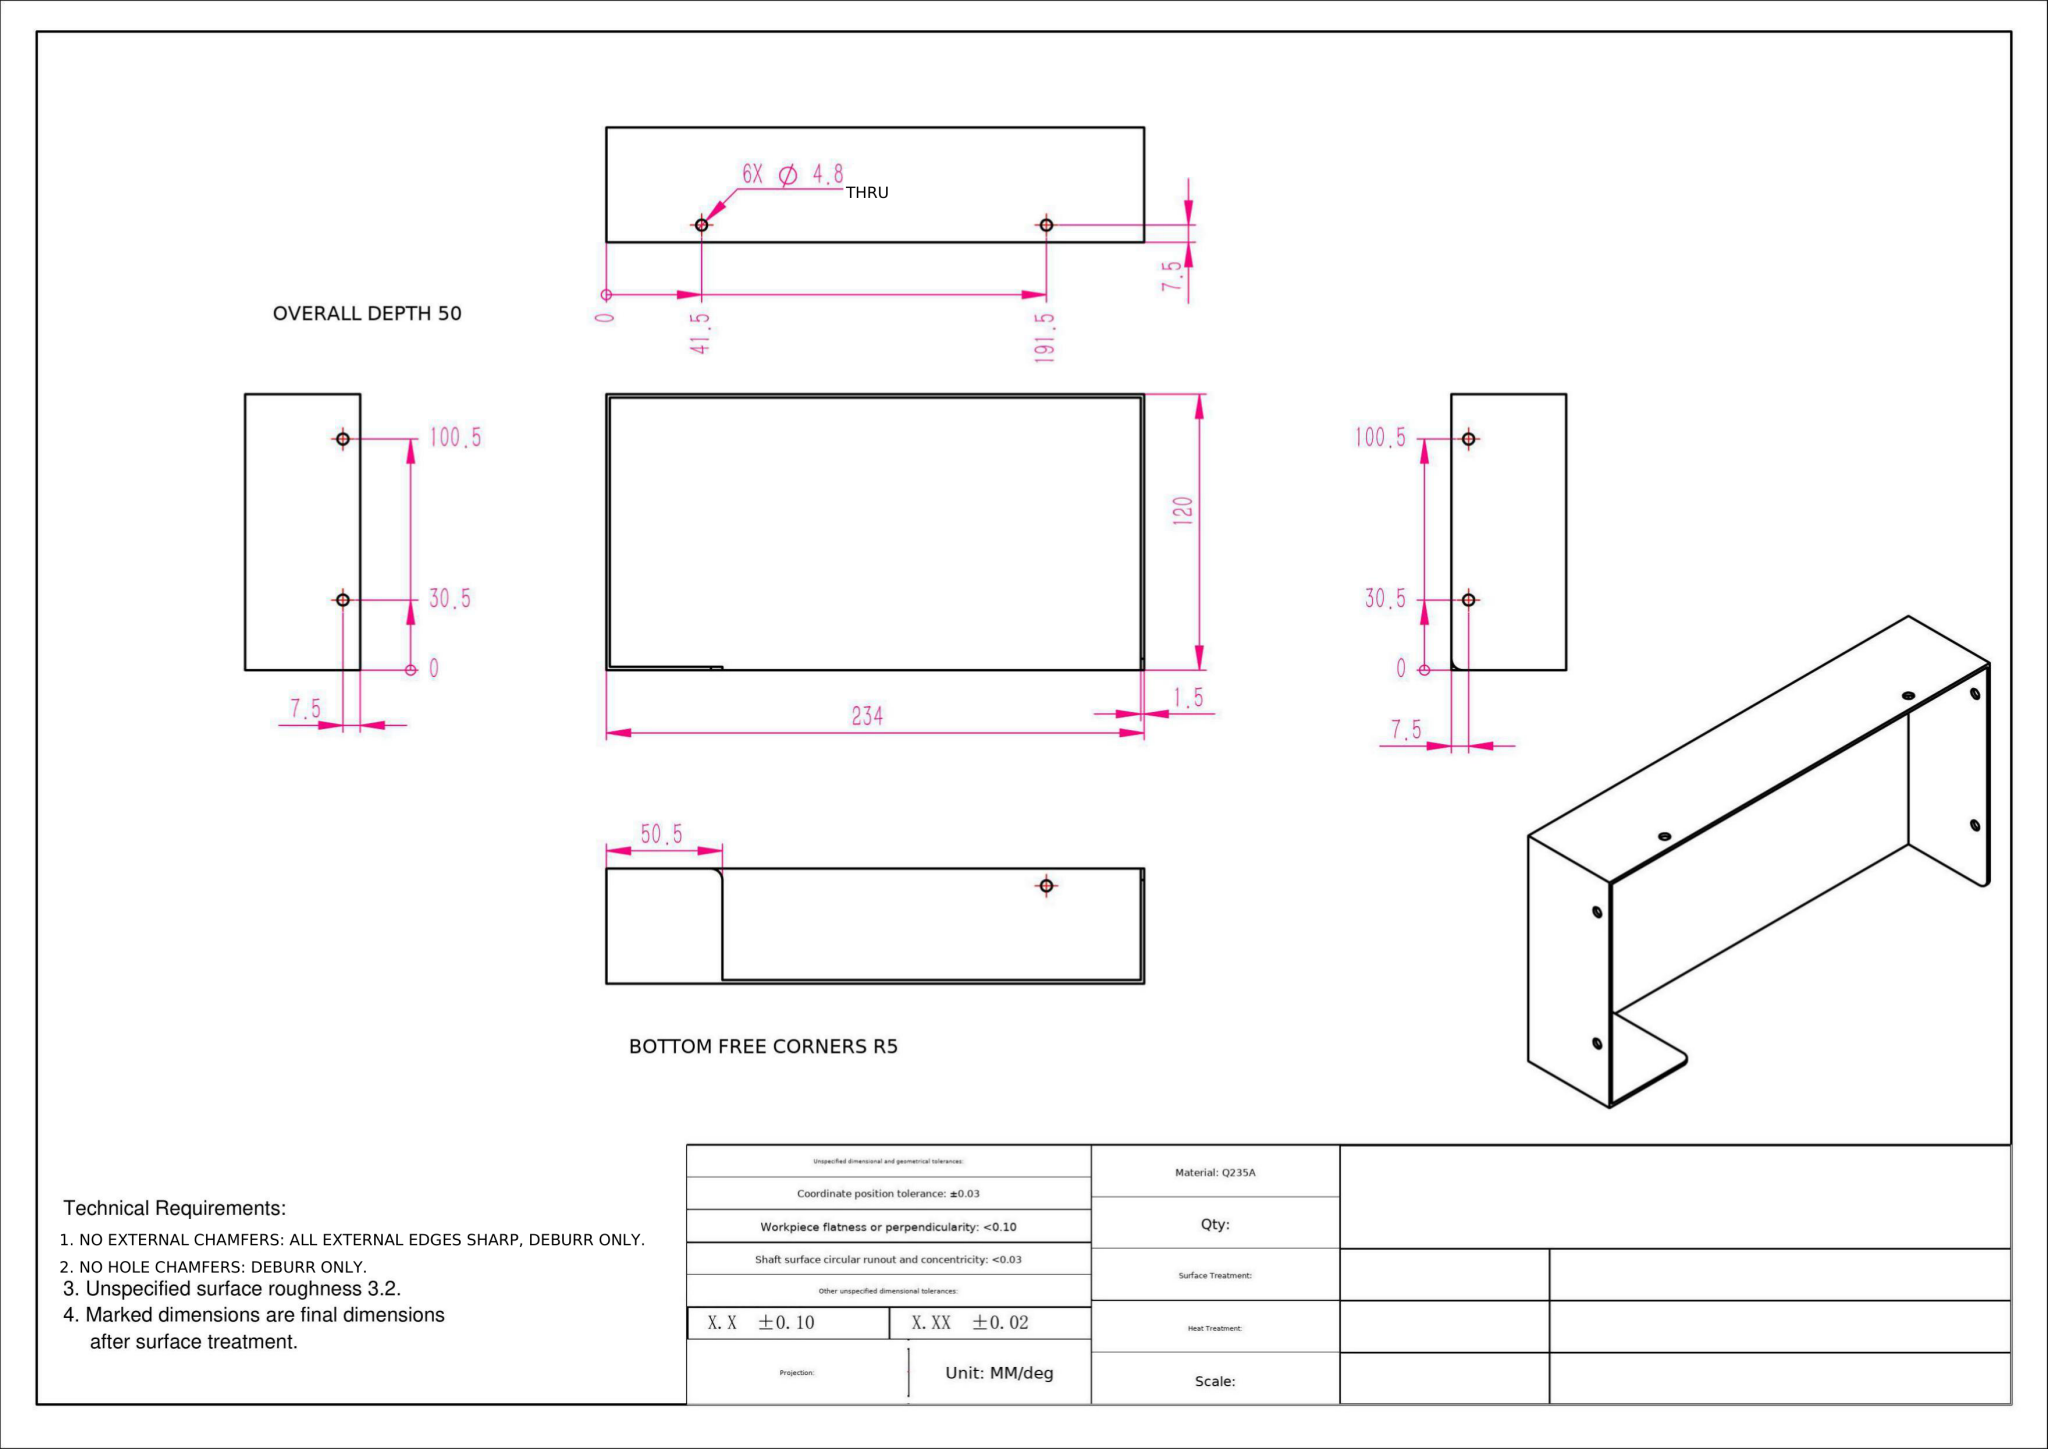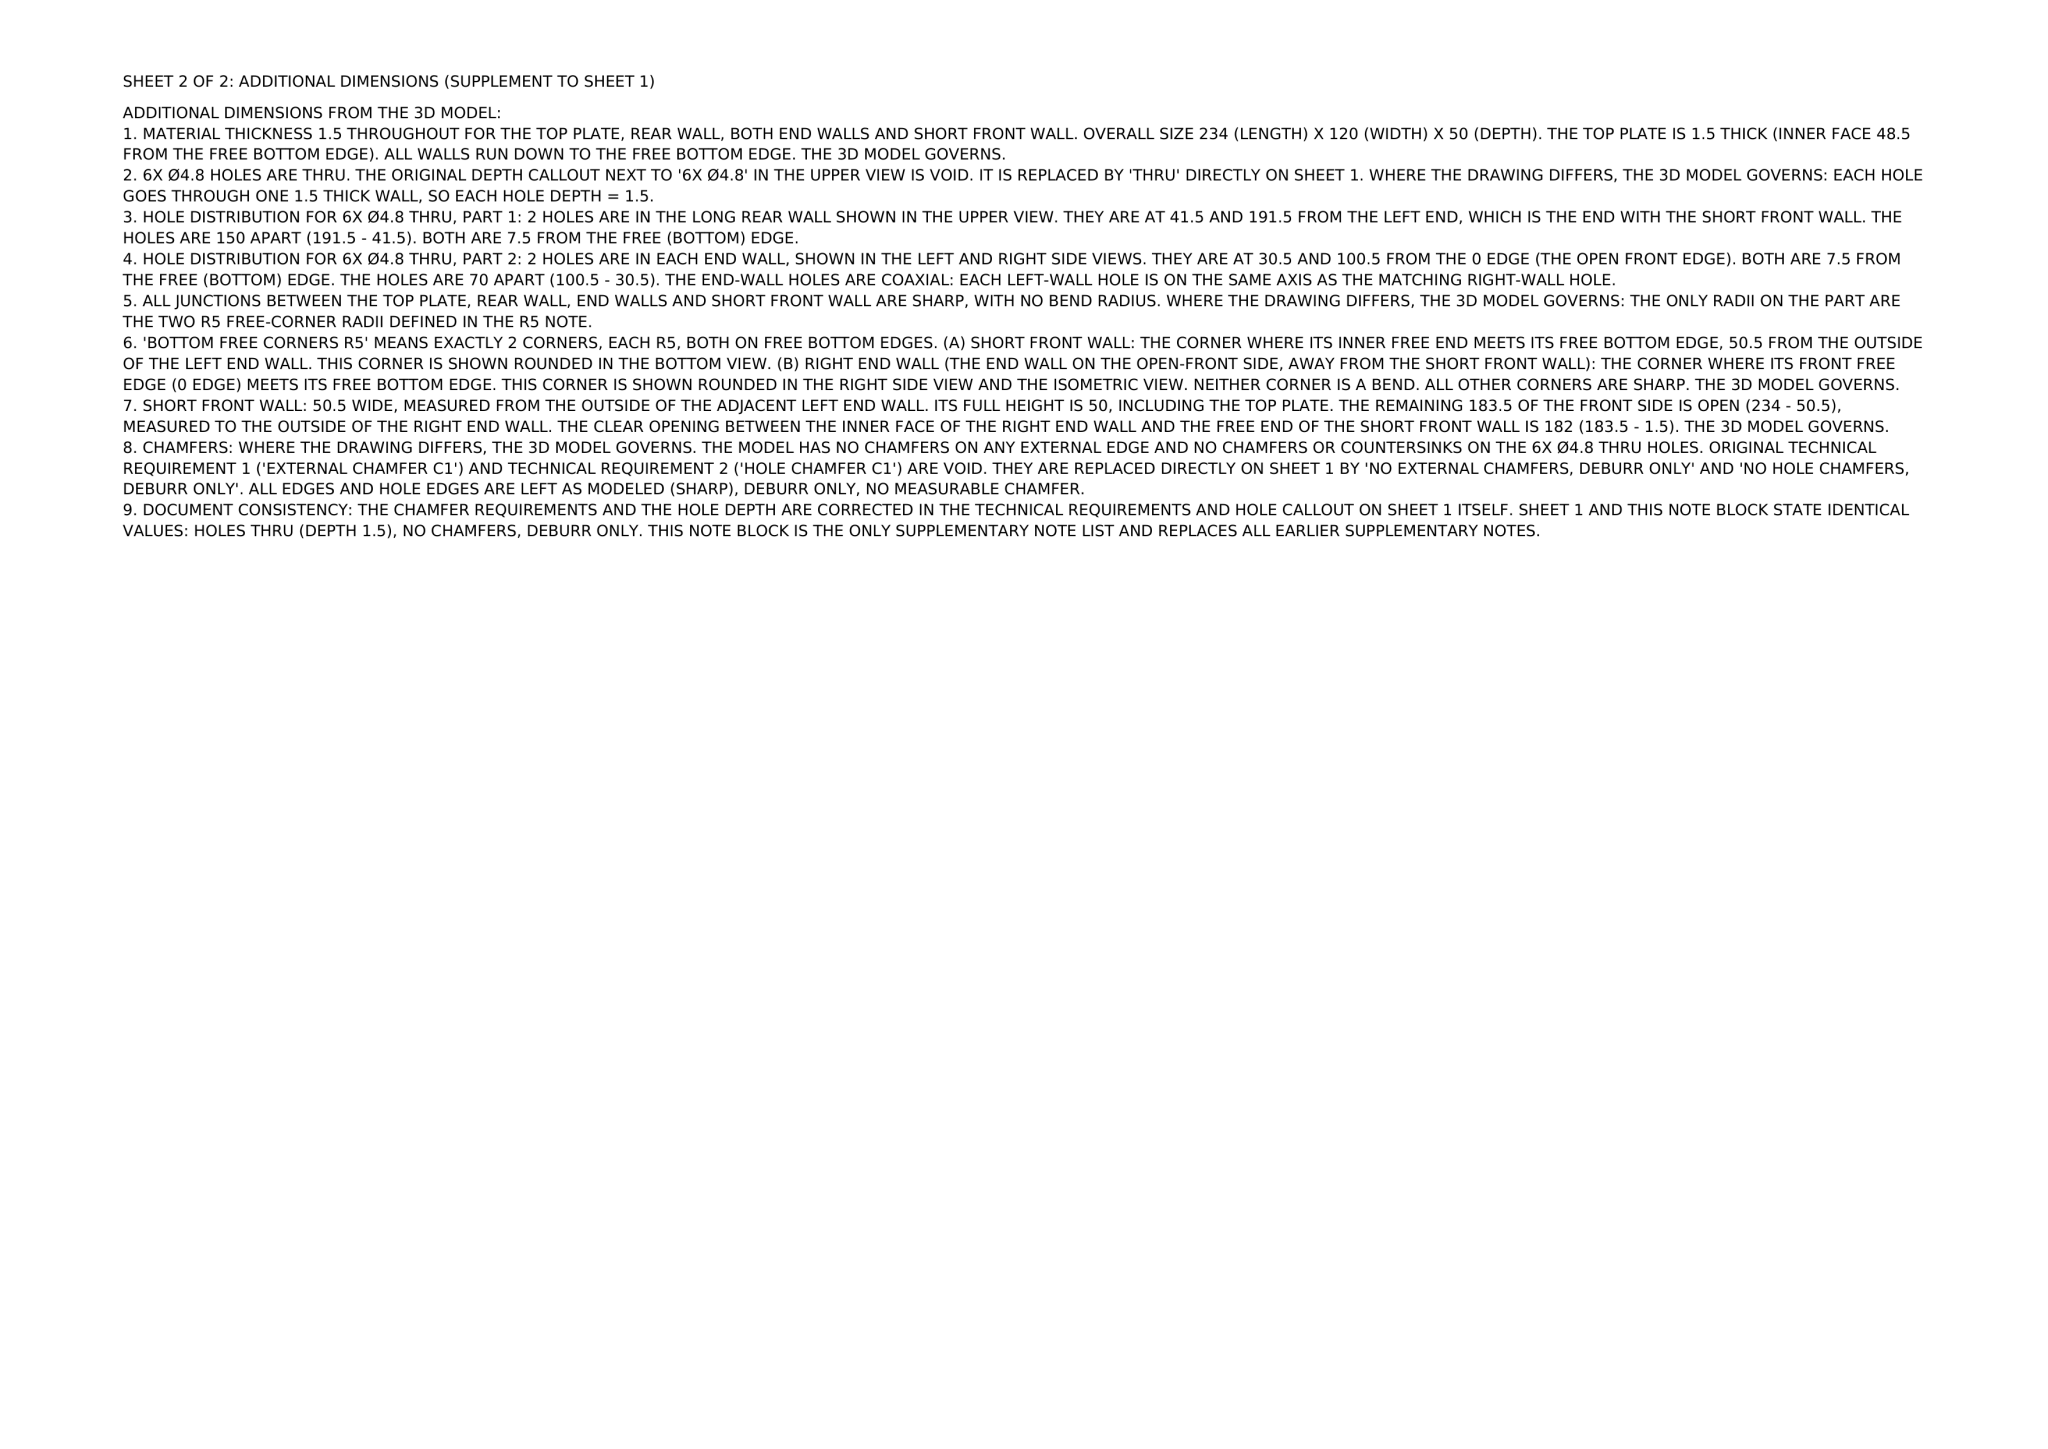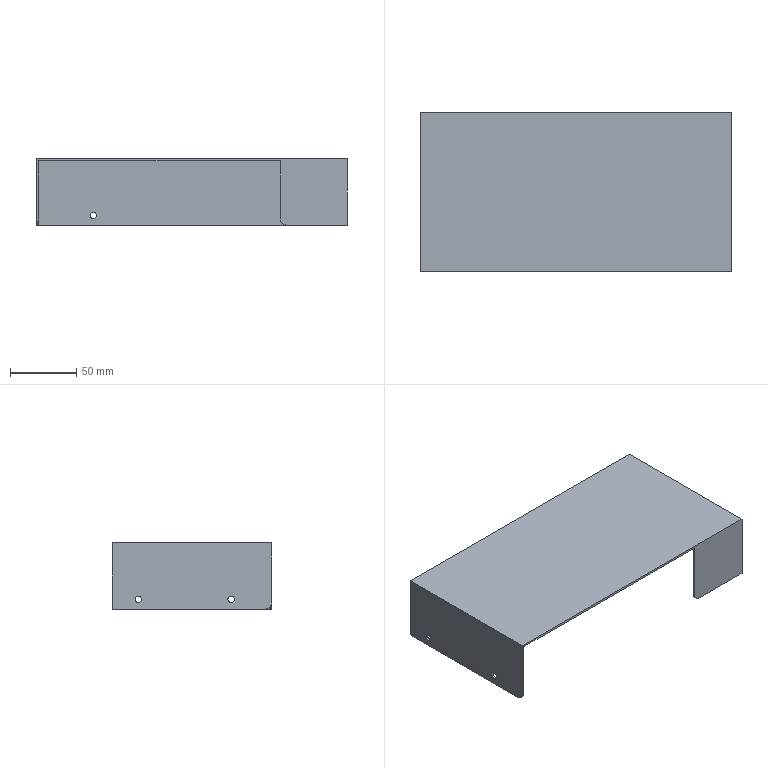Part | NX | mm | Rectangular U-Channel Frame Panel 120mm | 1 solid | 26 faces | box 234 x 120 x 50 mm | volume 79771 mm3 | cylinder 14 | plane 12 | commonest cylinder face diameters 4.8 x12 10 x2
STEP:
#1=COLOUR_RGB('',1.,1.,0.502);
#2=FILL_AREA_STYLE_COLOUR('',#1);
#3=FILL_AREA_STYLE('',(#2));
#4=SURFACE_STYLE_FILL_AREA(#3);
#5=SURFACE_SIDE_STYLE('',(#4));
#6=SURFACE_STYLE_USAGE(.BOTH.,#5);
#7=PRESENTATION_STYLE_ASSIGNMENT((#6));
#8=CARTESIAN_POINT('',(115.5,-29.5,5.1));
#9=VERTEX_POINT('',#8);
#10=CARTESIAN_POINT('',(115.5,-29.5,9.9));
#11=VERTEX_POINT('',#10);
#12=CARTESIAN_POINT('',(115.5,-29.5,7.5));
#13=DIRECTION('',(-1.,0.,0.));
#14=DIRECTION('',(0.,0.,1.));
#15=AXIS2_PLACEMENT_3D('',#12,#13,#14);
#16=CIRCLE('',#15,2.4);
#17=EDGE_CURVE('',#9,#11,#16,.T.);
#18=ORIENTED_EDGE('',*,*,#17,.T.);
#19=CARTESIAN_POINT('',(117.,-29.5,9.9));
#20=VERTEX_POINT('',#19);
#21=CARTESIAN_POINT('',(117.,-29.5,9.9));
#22=DIRECTION('',(1.,0.,0.));
#23=VECTOR('',#22,1000.);
#24=LINE('',#21,#23);
#25=EDGE_CURVE('',#11,#20,#24,.T.);
#26=ORIENTED_EDGE('',*,*,#25,.T.);
#27=CARTESIAN_POINT('',(117.,-29.5,5.1));
#28=VERTEX_POINT('',#27);
#29=CARTESIAN_POINT('',(117.,-29.5,7.5));
#30=DIRECTION('',(1.,0.,0.));
#31=DIRECTION('',(0.,0.,-1.));
#32=AXIS2_PLACEMENT_3D('',#29,#30,#31);
#33=CIRCLE('',#32,2.4);
#34=EDGE_CURVE('',#20,#28,#33,.T.);
#35=ORIENTED_EDGE('',*,*,#34,.T.);
#36=CARTESIAN_POINT('',(117.,-29.5,5.1));
#37=DIRECTION('',(1.,0.,0.));
#38=VECTOR('',#37,1000.);
#39=LINE('',#36,#38);
#40=EDGE_CURVE('',#9,#28,#39,.T.);
#41=ORIENTED_EDGE('',*,*,#40,.F.);
#42=EDGE_LOOP('',(#18,#26,#35,#41));
#43=FACE_OUTER_BOUND('',#42,.T.);
#44=CARTESIAN_POINT('',(117.,-29.5,7.5));
#45=DIRECTION('',(1.,0.,0.));
#46=DIRECTION('',(0.,0.,-1.));
#47=AXIS2_PLACEMENT_3D('',#44,#45,#46);
#48=CYLINDRICAL_SURFACE('',#47,2.4);
#49=ADVANCED_FACE('',(#43),#48,.F.);
#50=CARTESIAN_POINT('',(115.5,40.5,5.1));
#51=VERTEX_POINT('',#50);
#52=CARTESIAN_POINT('',(115.5,40.5,9.9));
#53=VERTEX_POINT('',#52);
#54=CARTESIAN_POINT('',(115.5,40.5,7.5));
#55=DIRECTION('',(-1.,0.,0.));
#56=DIRECTION('',(0.,0.,1.));
#57=AXIS2_PLACEMENT_3D('',#54,#55,#56);
#58=CIRCLE('',#57,2.4);
#59=EDGE_CURVE('',#51,#53,#58,.T.);
#60=ORIENTED_EDGE('',*,*,#59,.T.);
#61=CARTESIAN_POINT('',(117.,40.5,9.9));
#62=VERTEX_POINT('',#61);
#63=CARTESIAN_POINT('',(117.,40.5,9.9));
#64=DIRECTION('',(1.,0.,0.));
#65=VECTOR('',#64,1000.);
#66=LINE('',#63,#65);
#67=EDGE_CURVE('',#53,#62,#66,.T.);
#68=ORIENTED_EDGE('',*,*,#67,.T.);
#69=CARTESIAN_POINT('',(117.,40.5,5.1));
#70=VERTEX_POINT('',#69);
#71=CARTESIAN_POINT('',(117.,40.5,7.5));
#72=DIRECTION('',(1.,0.,0.));
#73=DIRECTION('',(0.,0.,-1.));
#74=AXIS2_PLACEMENT_3D('',#71,#72,#73);
#75=CIRCLE('',#74,2.4);
#76=EDGE_CURVE('',#62,#70,#75,.T.);
#77=ORIENTED_EDGE('',*,*,#76,.T.);
#78=CARTESIAN_POINT('',(117.,40.5,5.1));
#79=DIRECTION('',(1.,0.,0.));
#80=VECTOR('',#79,1000.);
#81=LINE('',#78,#80);
#82=EDGE_CURVE('',#51,#70,#81,.T.);
#83=ORIENTED_EDGE('',*,*,#82,.F.);
#84=EDGE_LOOP('',(#60,#68,#77,#83));
#85=FACE_OUTER_BOUND('',#84,.T.);
#86=CARTESIAN_POINT('',(117.,40.5,7.5));
#87=DIRECTION('',(1.,0.,0.));
#88=DIRECTION('',(0.,0.,-1.));
#89=AXIS2_PLACEMENT_3D('',#86,#87,#88);
#90=CYLINDRICAL_SURFACE('',#89,2.4);
#91=ADVANCED_FACE('',(#85),#90,.F.);
#92=CARTESIAN_POINT('',(75.5,58.5,9.9));
#93=VERTEX_POINT('',#92);
#94=CARTESIAN_POINT('',(75.5,58.5,5.1));
#95=VERTEX_POINT('',#94);
#96=CARTESIAN_POINT('',(75.5,58.5,7.5));
#97=DIRECTION('',(0.,-1.,0.));
#98=DIRECTION('',(0.,0.,-1.));
#99=AXIS2_PLACEMENT_3D('',#96,#97,#98);
#100=CIRCLE('',#99,2.4);
#101=EDGE_CURVE('',#93,#95,#100,.T.);
#102=ORIENTED_EDGE('',*,*,#101,.T.);
#103=CARTESIAN_POINT('',(75.5,60.,5.1));
#104=VERTEX_POINT('',#103);
#105=CARTESIAN_POINT('',(75.5,60.,5.1));
#106=DIRECTION('',(0.,1.,0.));
#107=VECTOR('',#106,1000.);
#108=LINE('',#105,#107);
#109=EDGE_CURVE('',#95,#104,#108,.T.);
#110=ORIENTED_EDGE('',*,*,#109,.T.);
#111=CARTESIAN_POINT('',(75.5,60.,9.9));
#112=VERTEX_POINT('',#111);
#113=CARTESIAN_POINT('',(75.5,60.,7.5));
#114=DIRECTION('',(0.,1.,0.));
#115=DIRECTION('',(0.,0.,1.));
#116=AXIS2_PLACEMENT_3D('',#113,#114,#115);
#117=CIRCLE('',#116,2.4);
#118=EDGE_CURVE('',#104,#112,#117,.T.);
#119=ORIENTED_EDGE('',*,*,#118,.T.);
#120=CARTESIAN_POINT('',(75.5,60.,9.9));
#121=DIRECTION('',(0.,1.,0.));
#122=VECTOR('',#121,1000.);
#123=LINE('',#120,#122);
#124=EDGE_CURVE('',#93,#112,#123,.T.);
#125=ORIENTED_EDGE('',*,*,#124,.F.);
#126=EDGE_LOOP('',(#102,#110,#119,#125));
#127=FACE_OUTER_BOUND('',#126,.T.);
#128=CARTESIAN_POINT('',(75.5,60.,7.5));
#129=DIRECTION('',(0.,1.,0.));
#130=DIRECTION('',(0.,0.,1.));
#131=AXIS2_PLACEMENT_3D('',#128,#129,#130);
#132=CYLINDRICAL_SURFACE('',#131,2.4);
#133=ADVANCED_FACE('',(#127),#132,.F.);
#134=CARTESIAN_POINT('',(-74.5,58.5,9.9));
#135=VERTEX_POINT('',#134);
#136=CARTESIAN_POINT('',(-74.5,58.5,5.1));
#137=VERTEX_POINT('',#136);
#138=CARTESIAN_POINT('',(-74.5,58.5,7.5));
#139=DIRECTION('',(0.,-1.,0.));
#140=DIRECTION('',(0.,0.,-1.));
#141=AXIS2_PLACEMENT_3D('',#138,#139,#140);
#142=CIRCLE('',#141,2.4);
#143=EDGE_CURVE('',#135,#137,#142,.T.);
#144=ORIENTED_EDGE('',*,*,#143,.T.);
#145=CARTESIAN_POINT('',(-74.5,60.,5.1));
#146=VERTEX_POINT('',#145);
#147=CARTESIAN_POINT('',(-74.5,60.,5.1));
#148=DIRECTION('',(0.,1.,0.));
#149=VECTOR('',#148,1000.);
#150=LINE('',#147,#149);
#151=EDGE_CURVE('',#137,#146,#150,.T.);
#152=ORIENTED_EDGE('',*,*,#151,.T.);
#153=CARTESIAN_POINT('',(-74.5,60.,9.9));
#154=VERTEX_POINT('',#153);
#155=CARTESIAN_POINT('',(-74.5,60.,7.5));
#156=DIRECTION('',(0.,1.,0.));
#157=DIRECTION('',(0.,0.,1.));
#158=AXIS2_PLACEMENT_3D('',#155,#156,#157);
#159=CIRCLE('',#158,2.4);
#160=EDGE_CURVE('',#146,#154,#159,.T.);
#161=ORIENTED_EDGE('',*,*,#160,.T.);
#162=CARTESIAN_POINT('',(-74.5,60.,9.9));
#163=DIRECTION('',(0.,1.,0.));
#164=VECTOR('',#163,1000.);
#165=LINE('',#162,#164);
#166=EDGE_CURVE('',#135,#154,#165,.T.);
#167=ORIENTED_EDGE('',*,*,#166,.F.);
#168=EDGE_LOOP('',(#144,#152,#161,#167));
#169=FACE_OUTER_BOUND('',#168,.T.);
#170=CARTESIAN_POINT('',(-74.5,60.,7.5));
#171=DIRECTION('',(0.,1.,0.));
#172=DIRECTION('',(0.,0.,1.));
#173=AXIS2_PLACEMENT_3D('',#170,#171,#172);
#174=CYLINDRICAL_SURFACE('',#173,2.4);
#175=ADVANCED_FACE('',(#169),#174,.F.);
#176=CARTESIAN_POINT('',(-115.5,40.5,9.9));
#177=VERTEX_POINT('',#176);
#178=CARTESIAN_POINT('',(-115.5,40.5,5.1));
#179=VERTEX_POINT('',#178);
#180=CARTESIAN_POINT('',(-115.5,40.5,7.5));
#181=DIRECTION('',(1.,0.,0.));
#182=DIRECTION('',(0.,0.,-1.));
#183=AXIS2_PLACEMENT_3D('',#180,#181,#182);
#184=CIRCLE('',#183,2.4);
#185=EDGE_CURVE('',#177,#179,#184,.T.);
#186=ORIENTED_EDGE('',*,*,#185,.T.);
#187=CARTESIAN_POINT('',(-117.,40.5,5.1));
#188=VERTEX_POINT('',#187);
#189=CARTESIAN_POINT('',(-117.,40.5,5.1));
#190=DIRECTION('',(-1.,0.,0.));
#191=VECTOR('',#190,1000.);
#192=LINE('',#189,#191);
#193=EDGE_CURVE('',#179,#188,#192,.T.);
#194=ORIENTED_EDGE('',*,*,#193,.T.);
#195=CARTESIAN_POINT('',(-117.,40.5,9.9));
#196=VERTEX_POINT('',#195);
#197=CARTESIAN_POINT('',(-117.,40.5,7.5));
#198=DIRECTION('',(-1.,0.,0.));
#199=DIRECTION('',(0.,0.,1.));
#200=AXIS2_PLACEMENT_3D('',#197,#198,#199);
#201=CIRCLE('',#200,2.4);
#202=EDGE_CURVE('',#188,#196,#201,.T.);
#203=ORIENTED_EDGE('',*,*,#202,.T.);
#204=CARTESIAN_POINT('',(-117.,40.5,9.9));
#205=DIRECTION('',(-1.,0.,0.));
#206=VECTOR('',#205,1000.);
#207=LINE('',#204,#206);
#208=EDGE_CURVE('',#177,#196,#207,.T.);
#209=ORIENTED_EDGE('',*,*,#208,.F.);
#210=EDGE_LOOP('',(#186,#194,#203,#209));
#211=FACE_OUTER_BOUND('',#210,.T.);
#212=CARTESIAN_POINT('',(-117.,40.5,7.5));
#213=DIRECTION('',(-1.,0.,0.));
#214=DIRECTION('',(0.,0.,1.));
#215=AXIS2_PLACEMENT_3D('',#212,#213,#214);
#216=CYLINDRICAL_SURFACE('',#215,2.4);
#217=ADVANCED_FACE('',(#211),#216,.F.);
#218=CARTESIAN_POINT('',(-115.5,-29.5,9.9));
#219=VERTEX_POINT('',#218);
#220=CARTESIAN_POINT('',(-115.5,-29.5,5.1));
#221=VERTEX_POINT('',#220);
#222=CARTESIAN_POINT('',(-115.5,-29.5,7.5));
#223=DIRECTION('',(1.,0.,0.));
#224=DIRECTION('',(0.,0.,-1.));
#225=AXIS2_PLACEMENT_3D('',#222,#223,#224);
#226=CIRCLE('',#225,2.4);
#227=EDGE_CURVE('',#219,#221,#226,.T.);
#228=ORIENTED_EDGE('',*,*,#227,.T.);
#229=CARTESIAN_POINT('',(-117.,-29.5,5.1));
#230=VERTEX_POINT('',#229);
#231=CARTESIAN_POINT('',(-117.,-29.5,5.1));
#232=DIRECTION('',(-1.,0.,0.));
#233=VECTOR('',#232,1000.);
#234=LINE('',#231,#233);
#235=EDGE_CURVE('',#221,#230,#234,.T.);
#236=ORIENTED_EDGE('',*,*,#235,.T.);
#237=CARTESIAN_POINT('',(-117.,-29.5,9.9));
#238=VERTEX_POINT('',#237);
#239=CARTESIAN_POINT('',(-117.,-29.5,7.5));
#240=DIRECTION('',(-1.,0.,0.));
#241=DIRECTION('',(0.,0.,1.));
#242=AXIS2_PLACEMENT_3D('',#239,#240,#241);
#243=CIRCLE('',#242,2.4);
#244=EDGE_CURVE('',#230,#238,#243,.T.);
#245=ORIENTED_EDGE('',*,*,#244,.T.);
#246=CARTESIAN_POINT('',(-117.,-29.5,9.9));
#247=DIRECTION('',(-1.,0.,0.));
#248=VECTOR('',#247,1000.);
#249=LINE('',#246,#248);
#250=EDGE_CURVE('',#219,#238,#249,.T.);
#251=ORIENTED_EDGE('',*,*,#250,.F.);
#252=EDGE_LOOP('',(#228,#236,#245,#251));
#253=FACE_OUTER_BOUND('',#252,.T.);
#254=CARTESIAN_POINT('',(-117.,-29.5,7.5));
#255=DIRECTION('',(-1.,0.,0.));
#256=DIRECTION('',(0.,0.,1.));
#257=AXIS2_PLACEMENT_3D('',#254,#255,#256);
#258=CYLINDRICAL_SURFACE('',#257,2.4);
#259=ADVANCED_FACE('',(#253),#258,.F.);
#260=CARTESIAN_POINT('',(71.5,-60.,0.));
#261=VERTEX_POINT('',#260);
#262=CARTESIAN_POINT('',(117.,-60.,0.));
#263=VERTEX_POINT('',#262);
#264=CARTESIAN_POINT('',(-117.,-60.,0.));
#265=DIRECTION('',(1.,0.,0.));
#266=VECTOR('',#265,1000.);
#267=LINE('',#264,#266);
#268=EDGE_CURVE('',#261,#263,#267,.T.);
#269=ORIENTED_EDGE('',*,*,#268,.F.);
#270=CARTESIAN_POINT('',(71.5,-58.5,0.));
#271=VERTEX_POINT('',#270);
#272=CARTESIAN_POINT('',(71.5,-58.5,0.));
#273=DIRECTION('',(0.,1.,0.));
#274=VECTOR('',#273,1000.);
#275=LINE('',#272,#274);
#276=EDGE_CURVE('',#261,#271,#275,.T.);
#277=ORIENTED_EDGE('',*,*,#276,.T.);
#278=CARTESIAN_POINT('',(115.5,-58.5,0.));
#279=VERTEX_POINT('',#278);
#280=CARTESIAN_POINT('',(0.,-58.5,0.));
#281=DIRECTION('',(1.,0.,0.));
#282=VECTOR('',#281,1000.);
#283=LINE('',#280,#282);
#284=EDGE_CURVE('',#271,#279,#283,.T.);
#285=ORIENTED_EDGE('',*,*,#284,.T.);
#286=CARTESIAN_POINT('',(115.5,58.5,0.));
#287=VERTEX_POINT('',#286);
#288=CARTESIAN_POINT('',(115.5,0.,0.));
#289=DIRECTION('',(0.,1.,0.));
#290=VECTOR('',#289,1000.);
#291=LINE('',#288,#290);
#292=EDGE_CURVE('',#279,#287,#291,.T.);
#293=ORIENTED_EDGE('',*,*,#292,.T.);
#294=CARTESIAN_POINT('',(-115.5,58.5,0.));
#295=VERTEX_POINT('',#294);
#296=CARTESIAN_POINT('',(0.,58.5,0.));
#297=DIRECTION('',(-1.,0.,0.));
#298=VECTOR('',#297,1000.);
#299=LINE('',#296,#298);
#300=EDGE_CURVE('',#287,#295,#299,.T.);
#301=ORIENTED_EDGE('',*,*,#300,.T.);
#302=CARTESIAN_POINT('',(-115.5,-55.,0.));
#303=VERTEX_POINT('',#302);
#304=CARTESIAN_POINT('',(-115.5,0.,0.));
#305=DIRECTION('',(0.,-1.,0.));
#306=VECTOR('',#305,1000.);
#307=LINE('',#304,#306);
#308=EDGE_CURVE('',#295,#303,#307,.T.);
#309=ORIENTED_EDGE('',*,*,#308,.T.);
#310=CARTESIAN_POINT('',(-117.,-55.,0.));
#311=VERTEX_POINT('',#310);
#312=CARTESIAN_POINT('',(-117.,-55.,0.));
#313=DIRECTION('',(-1.,0.,0.));
#314=VECTOR('',#313,1000.);
#315=LINE('',#312,#314);
#316=EDGE_CURVE('',#303,#311,#315,.T.);
#317=ORIENTED_EDGE('',*,*,#316,.T.);
#318=CARTESIAN_POINT('',(-117.,60.,0.));
#319=VERTEX_POINT('',#318);
#320=CARTESIAN_POINT('',(-117.,-60.,0.));
#321=DIRECTION('',(0.,-1.,0.));
#322=VECTOR('',#321,1000.);
#323=LINE('',#320,#322);
#324=EDGE_CURVE('',#319,#311,#323,.T.);
#325=ORIENTED_EDGE('',*,*,#324,.F.);
#326=CARTESIAN_POINT('',(117.,60.,0.));
#327=VERTEX_POINT('',#326);
#328=CARTESIAN_POINT('',(-117.,60.,0.));
#329=DIRECTION('',(-1.,0.,0.));
#330=VECTOR('',#329,1000.);
#331=LINE('',#328,#330);
#332=EDGE_CURVE('',#327,#319,#331,.T.);
#333=ORIENTED_EDGE('',*,*,#332,.F.);
#334=CARTESIAN_POINT('',(117.,-60.,0.));
#335=DIRECTION('',(0.,1.,0.));
#336=VECTOR('',#335,1000.);
#337=LINE('',#334,#336);
#338=EDGE_CURVE('',#263,#327,#337,.T.);
#339=ORIENTED_EDGE('',*,*,#338,.F.);
#340=EDGE_LOOP('',(#269,#277,#285,#293,#301,#309,#317,#325,#333,#339));
#341=FACE_OUTER_BOUND('',#340,.T.);
#342=CARTESIAN_POINT('',(0.,0.,0.));
#343=DIRECTION('',(0.,0.,-1.));
#344=DIRECTION('',(-1.,0.,0.));
#345=AXIS2_PLACEMENT_3D('',#342,#343,#344);
#346=PLANE('',#345);
#347=ADVANCED_FACE('',(#341),#346,.T.);
#348=CARTESIAN_POINT('',(117.,-29.5,7.5));
#349=DIRECTION('',(1.,0.,0.));
#350=DIRECTION('',(0.,0.,-1.));
#351=AXIS2_PLACEMENT_3D('',#348,#349,#350);
#352=CIRCLE('',#351,2.4);
#353=EDGE_CURVE('',#28,#20,#352,.T.);
#354=ORIENTED_EDGE('',*,*,#353,.F.);
#355=ORIENTED_EDGE('',*,*,#34,.F.);
#356=EDGE_LOOP('',(#354,#355));
#357=FACE_BOUND('',#356,.T.);
#358=CARTESIAN_POINT('',(117.,40.5,7.5));
#359=DIRECTION('',(1.,0.,0.));
#360=DIRECTION('',(0.,0.,-1.));
#361=AXIS2_PLACEMENT_3D('',#358,#359,#360);
#362=CIRCLE('',#361,2.4);
#363=EDGE_CURVE('',#70,#62,#362,.T.);
#364=ORIENTED_EDGE('',*,*,#363,.F.);
#365=ORIENTED_EDGE('',*,*,#76,.F.);
#366=EDGE_LOOP('',(#364,#365));
#367=FACE_BOUND('',#366,.T.);
#368=ORIENTED_EDGE('',*,*,#338,.T.);
#369=CARTESIAN_POINT('',(117.,60.,50.));
#370=VERTEX_POINT('',#369);
#371=CARTESIAN_POINT('',(117.,60.,50.));
#372=DIRECTION('',(0.,0.,-1.));
#373=VECTOR('',#372,1000.);
#374=LINE('',#371,#373);
#375=EDGE_CURVE('',#370,#327,#374,.T.);
#376=ORIENTED_EDGE('',*,*,#375,.F.);
#377=CARTESIAN_POINT('',(117.,-60.,50.));
#378=VERTEX_POINT('',#377);
#379=CARTESIAN_POINT('',(117.,-60.,50.));
#380=DIRECTION('',(0.,1.,0.));
#381=VECTOR('',#380,1000.);
#382=LINE('',#379,#381);
#383=EDGE_CURVE('',#378,#370,#382,.T.);
#384=ORIENTED_EDGE('',*,*,#383,.F.);
#385=CARTESIAN_POINT('',(117.,-60.,50.));
#386=DIRECTION('',(0.,0.,-1.));
#387=VECTOR('',#386,1000.);
#388=LINE('',#385,#387);
#389=EDGE_CURVE('',#378,#263,#388,.T.);
#390=ORIENTED_EDGE('',*,*,#389,.T.);
#391=EDGE_LOOP('',(#368,#376,#384,#390));
#392=FACE_OUTER_BOUND('',#391,.T.);
#393=CARTESIAN_POINT('',(117.,-60.,50.));
#394=DIRECTION('',(-1.,0.,0.));
#395=DIRECTION('',(0.,0.,1.));
#396=AXIS2_PLACEMENT_3D('',#393,#394,#395);
#397=PLANE('',#396);
#398=ADVANCED_FACE('',(#357,#367,#392),#397,.F.);
#399=CARTESIAN_POINT('',(75.5,60.,7.5));
#400=DIRECTION('',(0.,1.,0.));
#401=DIRECTION('',(0.,0.,1.));
#402=AXIS2_PLACEMENT_3D('',#399,#400,#401);
#403=CIRCLE('',#402,2.4);
#404=EDGE_CURVE('',#112,#104,#403,.T.);
#405=ORIENTED_EDGE('',*,*,#404,.F.);
#406=ORIENTED_EDGE('',*,*,#118,.F.);
#407=EDGE_LOOP('',(#405,#406));
#408=FACE_BOUND('',#407,.T.);
#409=CARTESIAN_POINT('',(-74.5,60.,7.5));
#410=DIRECTION('',(0.,1.,0.));
#411=DIRECTION('',(0.,0.,1.));
#412=AXIS2_PLACEMENT_3D('',#409,#410,#411);
#413=CIRCLE('',#412,2.4);
#414=EDGE_CURVE('',#154,#146,#413,.T.);
#415=ORIENTED_EDGE('',*,*,#414,.F.);
#416=ORIENTED_EDGE('',*,*,#160,.F.);
#417=EDGE_LOOP('',(#415,#416));
#418=FACE_BOUND('',#417,.T.);
#419=ORIENTED_EDGE('',*,*,#332,.T.);
#420=CARTESIAN_POINT('',(-117.,60.,50.));
#421=VERTEX_POINT('',#420);
#422=CARTESIAN_POINT('',(-117.,60.,50.));
#423=DIRECTION('',(0.,0.,-1.));
#424=VECTOR('',#423,1000.);
#425=LINE('',#422,#424);
#426=EDGE_CURVE('',#421,#319,#425,.T.);
#427=ORIENTED_EDGE('',*,*,#426,.F.);
#428=CARTESIAN_POINT('',(-117.,60.,50.));
#429=DIRECTION('',(-1.,0.,0.));
#430=VECTOR('',#429,1000.);
#431=LINE('',#428,#430);
#432=EDGE_CURVE('',#370,#421,#431,.T.);
#433=ORIENTED_EDGE('',*,*,#432,.F.);
#434=ORIENTED_EDGE('',*,*,#375,.T.);
#435=EDGE_LOOP('',(#419,#427,#433,#434));
#436=FACE_OUTER_BOUND('',#435,.T.);
#437=CARTESIAN_POINT('',(-117.,60.,50.));
#438=DIRECTION('',(0.,-1.,0.));
#439=DIRECTION('',(0.,0.,-1.));
#440=AXIS2_PLACEMENT_3D('',#437,#438,#439);
#441=PLANE('',#440);
#442=ADVANCED_FACE('',(#408,#418,#436),#441,.F.);
#443=CARTESIAN_POINT('',(-117.,40.5,7.5));
#444=DIRECTION('',(-1.,0.,0.));
#445=DIRECTION('',(0.,0.,1.));
#446=AXIS2_PLACEMENT_3D('',#443,#444,#445);
#447=CIRCLE('',#446,2.4);
#448=EDGE_CURVE('',#196,#188,#447,.T.);
#449=ORIENTED_EDGE('',*,*,#448,.F.);
#450=ORIENTED_EDGE('',*,*,#202,.F.);
#451=EDGE_LOOP('',(#449,#450));
#452=FACE_BOUND('',#451,.T.);
#453=CARTESIAN_POINT('',(-117.,-29.5,7.5));
#454=DIRECTION('',(-1.,0.,0.));
#455=DIRECTION('',(0.,0.,1.));
#456=AXIS2_PLACEMENT_3D('',#453,#454,#455);
#457=CIRCLE('',#456,2.4);
#458=EDGE_CURVE('',#238,#230,#457,.T.);
#459=ORIENTED_EDGE('',*,*,#458,.F.);
#460=ORIENTED_EDGE('',*,*,#244,.F.);
#461=EDGE_LOOP('',(#459,#460));
#462=FACE_BOUND('',#461,.T.);
#463=ORIENTED_EDGE('',*,*,#324,.T.);
#464=CARTESIAN_POINT('',(-117.,-60.,5.));
#465=VERTEX_POINT('',#464);
#466=CARTESIAN_POINT('',(-117.,-55.,5.));
#467=DIRECTION('',(-1.,0.,0.));
#468=DIRECTION('',(0.,0.,-1.));
#469=AXIS2_PLACEMENT_3D('',#466,#467,#468);
#470=CIRCLE('',#469,5.);
#471=EDGE_CURVE('',#311,#465,#470,.T.);
#472=ORIENTED_EDGE('',*,*,#471,.T.);
#473=CARTESIAN_POINT('',(-117.,-60.,50.));
#474=VERTEX_POINT('',#473);
#475=CARTESIAN_POINT('',(-117.,-60.,50.));
#476=DIRECTION('',(0.,0.,-1.));
#477=VECTOR('',#476,1000.);
#478=LINE('',#475,#477);
#479=EDGE_CURVE('',#474,#465,#478,.T.);
#480=ORIENTED_EDGE('',*,*,#479,.F.);
#481=CARTESIAN_POINT('',(-117.,-60.,50.));
#482=DIRECTION('',(0.,-1.,0.));
#483=VECTOR('',#482,1000.);
#484=LINE('',#481,#483);
#485=EDGE_CURVE('',#421,#474,#484,.T.);
#486=ORIENTED_EDGE('',*,*,#485,.F.);
#487=ORIENTED_EDGE('',*,*,#426,.T.);
#488=EDGE_LOOP('',(#463,#472,#480,#486,#487));
#489=FACE_OUTER_BOUND('',#488,.T.);
#490=CARTESIAN_POINT('',(-117.,-60.,50.));
#491=DIRECTION('',(1.,0.,0.));
#492=DIRECTION('',(0.,0.,-1.));
#493=AXIS2_PLACEMENT_3D('',#490,#491,#492);
#494=PLANE('',#493);
#495=ADVANCED_FACE('',(#452,#462,#489),#494,.F.);
#496=CARTESIAN_POINT('',(66.5,-60.,5.));
#497=VERTEX_POINT('',#496);
#498=CARTESIAN_POINT('',(66.5,-60.,48.5));
#499=VERTEX_POINT('',#498);
#500=CARTESIAN_POINT('',(66.5,-60.,0.));
#501=DIRECTION('',(0.,0.,1.));
#502=VECTOR('',#501,1000.);
#503=LINE('',#500,#502);
#504=EDGE_CURVE('',#497,#499,#503,.T.);
#505=ORIENTED_EDGE('',*,*,#504,.F.);
#506=CARTESIAN_POINT('',(71.5,-60.,5.));
#507=DIRECTION('',(0.,-1.,0.));
#508=DIRECTION('',(0.,0.,1.));
#509=AXIS2_PLACEMENT_3D('',#506,#507,#508);
#510=CIRCLE('',#509,5.);
#511=EDGE_CURVE('',#497,#261,#510,.T.);
#512=ORIENTED_EDGE('',*,*,#511,.T.);
#513=ORIENTED_EDGE('',*,*,#268,.T.);
#514=ORIENTED_EDGE('',*,*,#389,.F.);
#515=CARTESIAN_POINT('',(-117.,-60.,50.));
#516=DIRECTION('',(1.,0.,0.));
#517=VECTOR('',#516,1000.);
#518=LINE('',#515,#517);
#519=EDGE_CURVE('',#474,#378,#518,.T.);
#520=ORIENTED_EDGE('',*,*,#519,.F.);
#521=ORIENTED_EDGE('',*,*,#479,.T.);
#522=CARTESIAN_POINT('',(-115.5,-60.,5.));
#523=VERTEX_POINT('',#522);
#524=CARTESIAN_POINT('',(-115.5,-60.,5.));
#525=DIRECTION('',(1.,0.,0.));
#526=VECTOR('',#525,1000.);
#527=LINE('',#524,#526);
#528=EDGE_CURVE('',#465,#523,#527,.T.);
#529=ORIENTED_EDGE('',*,*,#528,.T.);
#530=CARTESIAN_POINT('',(-115.5,-60.,48.5));
#531=VERTEX_POINT('',#530);
#532=CARTESIAN_POINT('',(-115.5,-60.,-0.));
#533=DIRECTION('',(0.,0.,-1.));
#534=VECTOR('',#533,1000.);
#535=LINE('',#532,#534);
#536=EDGE_CURVE('',#531,#523,#535,.T.);
#537=ORIENTED_EDGE('',*,*,#536,.F.);
#538=CARTESIAN_POINT('',(66.5,-60.,48.5));
#539=DIRECTION('',(-1.,0.,-0.));
#540=VECTOR('',#539,1000.);
#541=LINE('',#538,#540);
#542=EDGE_CURVE('',#499,#531,#541,.T.);
#543=ORIENTED_EDGE('',*,*,#542,.F.);
#544=EDGE_LOOP('',(#505,#512,#513,#514,#520,#521,#529,#537,#543));
#545=FACE_OUTER_BOUND('',#544,.T.);
#546=CARTESIAN_POINT('',(-117.,-60.,50.));
#547=DIRECTION('',(0.,1.,0.));
#548=DIRECTION('',(0.,0.,1.));
#549=AXIS2_PLACEMENT_3D('',#546,#547,#548);
#550=PLANE('',#549);
#551=ADVANCED_FACE('',(#545),#550,.F.);
#552=ORIENTED_EDGE('',*,*,#383,.T.);
#553=ORIENTED_EDGE('',*,*,#432,.T.);
#554=ORIENTED_EDGE('',*,*,#485,.T.);
#555=ORIENTED_EDGE('',*,*,#519,.T.);
#556=EDGE_LOOP('',(#552,#553,#554,#555));
#557=FACE_OUTER_BOUND('',#556,.T.);
#558=CARTESIAN_POINT('',(0.,0.,50.));
#559=DIRECTION('',(0.,0.,-1.));
#560=DIRECTION('',(-1.,0.,0.));
#561=AXIS2_PLACEMENT_3D('',#558,#559,#560);
#562=PLANE('',#561);
#563=ADVANCED_FACE('',(#557),#562,.F.);
#564=ORIENTED_EDGE('',*,*,#17,.F.);
#565=CARTESIAN_POINT('',(115.5,-29.5,7.5));
#566=DIRECTION('',(-1.,0.,0.));
#567=DIRECTION('',(0.,0.,1.));
#568=AXIS2_PLACEMENT_3D('',#565,#566,#567);
#569=CIRCLE('',#568,2.4);
#570=EDGE_CURVE('',#11,#9,#569,.T.);
#571=ORIENTED_EDGE('',*,*,#570,.F.);
#572=EDGE_LOOP('',(#564,#571));
#573=FACE_BOUND('',#572,.T.);
#574=ORIENTED_EDGE('',*,*,#59,.F.);
#575=CARTESIAN_POINT('',(115.5,40.5,7.5));
#576=DIRECTION('',(-1.,0.,0.));
#577=DIRECTION('',(0.,0.,1.));
#578=AXIS2_PLACEMENT_3D('',#575,#576,#577);
#579=CIRCLE('',#578,2.4);
#580=EDGE_CURVE('',#53,#51,#579,.T.);
#581=ORIENTED_EDGE('',*,*,#580,.F.);
#582=EDGE_LOOP('',(#574,#581));
#583=FACE_BOUND('',#582,.T.);
#584=ORIENTED_EDGE('',*,*,#292,.F.);
#585=CARTESIAN_POINT('',(115.5,-58.5,48.5));
#586=VERTEX_POINT('',#585);
#587=CARTESIAN_POINT('',(115.5,-58.5,50.));
#588=DIRECTION('',(0.,0.,-1.));
#589=VECTOR('',#588,1000.);
#590=LINE('',#587,#589);
#591=EDGE_CURVE('',#586,#279,#590,.T.);
#592=ORIENTED_EDGE('',*,*,#591,.F.);
#593=CARTESIAN_POINT('',(115.5,58.5,48.5));
#594=VERTEX_POINT('',#593);
#595=CARTESIAN_POINT('',(115.5,0.,48.5));
#596=DIRECTION('',(0.,1.,0.));
#597=VECTOR('',#596,1000.);
#598=LINE('',#595,#597);
#599=EDGE_CURVE('',#586,#594,#598,.T.);
#600=ORIENTED_EDGE('',*,*,#599,.T.);
#601=CARTESIAN_POINT('',(115.5,58.5,50.));
#602=DIRECTION('',(0.,0.,-1.));
#603=VECTOR('',#602,1000.);
#604=LINE('',#601,#603);
#605=EDGE_CURVE('',#594,#287,#604,.T.);
#606=ORIENTED_EDGE('',*,*,#605,.T.);
#607=EDGE_LOOP('',(#584,#592,#600,#606));
#608=FACE_OUTER_BOUND('',#607,.T.);
#609=CARTESIAN_POINT('',(115.5,-60.,50.));
#610=DIRECTION('',(-1.,0.,0.));
#611=DIRECTION('',(0.,0.,1.));
#612=AXIS2_PLACEMENT_3D('',#609,#610,#611);
#613=PLANE('',#612);
#614=ADVANCED_FACE('',(#573,#583,#608),#613,.T.);
#615=ORIENTED_EDGE('',*,*,#101,.F.);
#616=CARTESIAN_POINT('',(75.5,58.5,7.5));
#617=DIRECTION('',(0.,-1.,0.));
#618=DIRECTION('',(0.,0.,-1.));
#619=AXIS2_PLACEMENT_3D('',#616,#617,#618);
#620=CIRCLE('',#619,2.4);
#621=EDGE_CURVE('',#95,#93,#620,.T.);
#622=ORIENTED_EDGE('',*,*,#621,.F.);
#623=EDGE_LOOP('',(#615,#622));
#624=FACE_BOUND('',#623,.T.);
#625=ORIENTED_EDGE('',*,*,#143,.F.);
#626=CARTESIAN_POINT('',(-74.5,58.5,7.5));
#627=DIRECTION('',(0.,-1.,0.));
#628=DIRECTION('',(0.,0.,-1.));
#629=AXIS2_PLACEMENT_3D('',#626,#627,#628);
#630=CIRCLE('',#629,2.4);
#631=EDGE_CURVE('',#137,#135,#630,.T.);
#632=ORIENTED_EDGE('',*,*,#631,.F.);
#633=EDGE_LOOP('',(#625,#632));
#634=FACE_BOUND('',#633,.T.);
#635=ORIENTED_EDGE('',*,*,#300,.F.);
#636=ORIENTED_EDGE('',*,*,#605,.F.);
#637=CARTESIAN_POINT('',(-115.5,58.5,48.5));
#638=VERTEX_POINT('',#637);
#639=CARTESIAN_POINT('',(0.,58.5,48.5));
#640=DIRECTION('',(-1.,0.,0.));
#641=VECTOR('',#640,1000.);
#642=LINE('',#639,#641);
#643=EDGE_CURVE('',#594,#638,#642,.T.);
#644=ORIENTED_EDGE('',*,*,#643,.T.);
#645=CARTESIAN_POINT('',(-115.5,58.5,50.));
#646=DIRECTION('',(0.,0.,-1.));
#647=VECTOR('',#646,1000.);
#648=LINE('',#645,#647);
#649=EDGE_CURVE('',#638,#295,#648,.T.);
#650=ORIENTED_EDGE('',*,*,#649,.T.);
#651=EDGE_LOOP('',(#635,#636,#644,#650));
#652=FACE_OUTER_BOUND('',#651,.T.);
#653=CARTESIAN_POINT('',(-117.,58.5,50.));
#654=DIRECTION('',(0.,-1.,0.));
#655=DIRECTION('',(0.,0.,-1.));
#656=AXIS2_PLACEMENT_3D('',#653,#654,#655);
#657=PLANE('',#656);
#658=ADVANCED_FACE('',(#624,#634,#652),#657,.T.);
#659=ORIENTED_EDGE('',*,*,#185,.F.);
#660=CARTESIAN_POINT('',(-115.5,40.5,7.5));
#661=DIRECTION('',(1.,0.,0.));
#662=DIRECTION('',(0.,0.,-1.));
#663=AXIS2_PLACEMENT_3D('',#660,#661,#662);
#664=CIRCLE('',#663,2.4);
#665=EDGE_CURVE('',#179,#177,#664,.T.);
#666=ORIENTED_EDGE('',*,*,#665,.F.);
#667=EDGE_LOOP('',(#659,#666));
#668=FACE_BOUND('',#667,.T.);
#669=ORIENTED_EDGE('',*,*,#227,.F.);
#670=CARTESIAN_POINT('',(-115.5,-29.5,7.5));
#671=DIRECTION('',(1.,0.,0.));
#672=DIRECTION('',(0.,0.,-1.));
#673=AXIS2_PLACEMENT_3D('',#670,#671,#672);
#674=CIRCLE('',#673,2.4);
#675=EDGE_CURVE('',#221,#219,#674,.T.);
#676=ORIENTED_EDGE('',*,*,#675,.F.);
#677=EDGE_LOOP('',(#669,#676));
#678=FACE_BOUND('',#677,.T.);
#679=ORIENTED_EDGE('',*,*,#536,.T.);
#680=CARTESIAN_POINT('',(-115.5,-55.,5.));
#681=DIRECTION('',(1.,0.,0.));
#682=DIRECTION('',(0.,0.,-1.));
#683=AXIS2_PLACEMENT_3D('',#680,#681,#682);
#684=CIRCLE('',#683,5.);
#685=EDGE_CURVE('',#523,#303,#684,.T.);
#686=ORIENTED_EDGE('',*,*,#685,.T.);
#687=ORIENTED_EDGE('',*,*,#308,.F.);
#688=ORIENTED_EDGE('',*,*,#649,.F.);
#689=CARTESIAN_POINT('',(-115.5,0.,48.5));
#690=DIRECTION('',(0.,-1.,0.));
#691=VECTOR('',#690,1000.);
#692=LINE('',#689,#691);
#693=EDGE_CURVE('',#638,#531,#692,.T.);
#694=ORIENTED_EDGE('',*,*,#693,.T.);
#695=EDGE_LOOP('',(#679,#686,#687,#688,#694));
#696=FACE_OUTER_BOUND('',#695,.T.);
#697=CARTESIAN_POINT('',(-115.5,-60.,50.));
#698=DIRECTION('',(1.,0.,0.));
#699=DIRECTION('',(0.,0.,-1.));
#700=AXIS2_PLACEMENT_3D('',#697,#698,#699);
#701=PLANE('',#700);
#702=ADVANCED_FACE('',(#668,#678,#696),#701,.T.);
#703=ORIENTED_EDGE('',*,*,#284,.F.);
#704=CARTESIAN_POINT('',(66.5,-58.5,5.));
#705=VERTEX_POINT('',#704);
#706=CARTESIAN_POINT('',(71.5,-58.5,5.));
#707=DIRECTION('',(0.,1.,0.));
#708=DIRECTION('',(0.,0.,1.));
#709=AXIS2_PLACEMENT_3D('',#706,#707,#708);
#710=CIRCLE('',#709,5.);
#711=EDGE_CURVE('',#271,#705,#710,.T.);
#712=ORIENTED_EDGE('',*,*,#711,.T.);
#713=CARTESIAN_POINT('',(66.5,-58.5,48.5));
#714=VERTEX_POINT('',#713);
#715=CARTESIAN_POINT('',(66.5,-58.5,0.));
#716=DIRECTION('',(0.,0.,1.));
#717=VECTOR('',#716,1000.);
#718=LINE('',#715,#717);
#719=EDGE_CURVE('',#705,#714,#718,.T.);
#720=ORIENTED_EDGE('',*,*,#719,.T.);
#721=CARTESIAN_POINT('',(0.,-58.5,48.5));
#722=DIRECTION('',(1.,0.,0.));
#723=VECTOR('',#722,1000.);
#724=LINE('',#721,#723);
#725=EDGE_CURVE('',#714,#586,#724,.T.);
#726=ORIENTED_EDGE('',*,*,#725,.T.);
#727=ORIENTED_EDGE('',*,*,#591,.T.);
#728=EDGE_LOOP('',(#703,#712,#720,#726,#727));
#729=FACE_OUTER_BOUND('',#728,.T.);
#730=CARTESIAN_POINT('',(-117.,-58.5,50.));
#731=DIRECTION('',(0.,1.,0.));
#732=DIRECTION('',(0.,0.,1.));
#733=AXIS2_PLACEMENT_3D('',#730,#731,#732);
#734=PLANE('',#733);
#735=ADVANCED_FACE('',(#729),#734,.T.);
#736=ORIENTED_EDGE('',*,*,#599,.F.);
#737=ORIENTED_EDGE('',*,*,#725,.F.);
#738=CARTESIAN_POINT('',(66.5,129.851,48.5));
#739=DIRECTION('',(0.,-1.,0.));
#740=VECTOR('',#739,1000.);
#741=LINE('',#738,#740);
#742=EDGE_CURVE('',#714,#499,#741,.T.);
#743=ORIENTED_EDGE('',*,*,#742,.T.);
#744=ORIENTED_EDGE('',*,*,#542,.T.);
#745=ORIENTED_EDGE('',*,*,#693,.F.);
#746=ORIENTED_EDGE('',*,*,#643,.F.);
#747=EDGE_LOOP('',(#736,#737,#743,#744,#745,#746));
#748=FACE_OUTER_BOUND('',#747,.T.);
#749=CARTESIAN_POINT('',(0.,0.,48.5));
#750=DIRECTION('',(0.,0.,-1.));
#751=DIRECTION('',(-1.,0.,0.));
#752=AXIS2_PLACEMENT_3D('',#749,#750,#751);
#753=PLANE('',#752);
#754=ADVANCED_FACE('',(#748),#753,.T.);
#755=ORIENTED_EDGE('',*,*,#719,.F.);
#756=CARTESIAN_POINT('',(66.5,-60.,5.));
#757=DIRECTION('',(0.,-1.,0.));
#758=VECTOR('',#757,1000.);
#759=LINE('',#756,#758);
#760=EDGE_CURVE('',#705,#497,#759,.T.);
#761=ORIENTED_EDGE('',*,*,#760,.T.);
#762=ORIENTED_EDGE('',*,*,#504,.T.);
#763=ORIENTED_EDGE('',*,*,#742,.F.);
#764=EDGE_LOOP('',(#755,#761,#762,#763));
#765=FACE_OUTER_BOUND('',#764,.T.);
#766=CARTESIAN_POINT('',(66.5,129.851,0.));
#767=DIRECTION('',(1.,0.,0.));
#768=DIRECTION('',(0.,0.,-1.));
#769=AXIS2_PLACEMENT_3D('',#766,#767,#768);
#770=PLANE('',#769);
#771=ADVANCED_FACE('',(#765),#770,.F.);
#772=ORIENTED_EDGE('',*,*,#235,.F.);
#773=ORIENTED_EDGE('',*,*,#675,.T.);
#774=ORIENTED_EDGE('',*,*,#250,.T.);
#775=ORIENTED_EDGE('',*,*,#458,.T.);
#776=EDGE_LOOP('',(#772,#773,#774,#775));
#777=FACE_OUTER_BOUND('',#776,.T.);
#778=CARTESIAN_POINT('',(-117.,-29.5,7.5));
#779=DIRECTION('',(-1.,0.,0.));
#780=DIRECTION('',(0.,0.,1.));
#781=AXIS2_PLACEMENT_3D('',#778,#779,#780);
#782=CYLINDRICAL_SURFACE('',#781,2.4);
#783=ADVANCED_FACE('',(#777),#782,.F.);
#784=ORIENTED_EDGE('',*,*,#193,.F.);
#785=ORIENTED_EDGE('',*,*,#665,.T.);
#786=ORIENTED_EDGE('',*,*,#208,.T.);
#787=ORIENTED_EDGE('',*,*,#448,.T.);
#788=EDGE_LOOP('',(#784,#785,#786,#787));
#789=FACE_OUTER_BOUND('',#788,.T.);
#790=CARTESIAN_POINT('',(-117.,40.5,7.5));
#791=DIRECTION('',(-1.,0.,0.));
#792=DIRECTION('',(0.,0.,1.));
#793=AXIS2_PLACEMENT_3D('',#790,#791,#792);
#794=CYLINDRICAL_SURFACE('',#793,2.4);
#795=ADVANCED_FACE('',(#789),#794,.F.);
#796=ORIENTED_EDGE('',*,*,#151,.F.);
#797=ORIENTED_EDGE('',*,*,#631,.T.);
#798=ORIENTED_EDGE('',*,*,#166,.T.);
#799=ORIENTED_EDGE('',*,*,#414,.T.);
#800=EDGE_LOOP('',(#796,#797,#798,#799));
#801=FACE_OUTER_BOUND('',#800,.T.);
#802=CARTESIAN_POINT('',(-74.5,60.,7.5));
#803=DIRECTION('',(0.,1.,0.));
#804=DIRECTION('',(0.,0.,1.));
#805=AXIS2_PLACEMENT_3D('',#802,#803,#804);
#806=CYLINDRICAL_SURFACE('',#805,2.4);
#807=ADVANCED_FACE('',(#801),#806,.F.);
#808=ORIENTED_EDGE('',*,*,#109,.F.);
#809=ORIENTED_EDGE('',*,*,#621,.T.);
#810=ORIENTED_EDGE('',*,*,#124,.T.);
#811=ORIENTED_EDGE('',*,*,#404,.T.);
#812=EDGE_LOOP('',(#808,#809,#810,#811));
#813=FACE_OUTER_BOUND('',#812,.T.);
#814=CARTESIAN_POINT('',(75.5,60.,7.5));
#815=DIRECTION('',(0.,1.,0.));
#816=DIRECTION('',(0.,0.,1.));
#817=AXIS2_PLACEMENT_3D('',#814,#815,#816);
#818=CYLINDRICAL_SURFACE('',#817,2.4);
#819=ADVANCED_FACE('',(#813),#818,.F.);
#820=ORIENTED_EDGE('',*,*,#67,.F.);
#821=ORIENTED_EDGE('',*,*,#580,.T.);
#822=ORIENTED_EDGE('',*,*,#82,.T.);
#823=ORIENTED_EDGE('',*,*,#363,.T.);
#824=EDGE_LOOP('',(#820,#821,#822,#823));
#825=FACE_OUTER_BOUND('',#824,.T.);
#826=CARTESIAN_POINT('',(117.,40.5,7.5));
#827=DIRECTION('',(1.,0.,0.));
#828=DIRECTION('',(0.,0.,-1.));
#829=AXIS2_PLACEMENT_3D('',#826,#827,#828);
#830=CYLINDRICAL_SURFACE('',#829,2.4);
#831=ADVANCED_FACE('',(#825),#830,.F.);
#832=ORIENTED_EDGE('',*,*,#25,.F.);
#833=ORIENTED_EDGE('',*,*,#570,.T.);
#834=ORIENTED_EDGE('',*,*,#40,.T.);
#835=ORIENTED_EDGE('',*,*,#353,.T.);
#836=EDGE_LOOP('',(#832,#833,#834,#835));
#837=FACE_OUTER_BOUND('',#836,.T.);
#838=CARTESIAN_POINT('',(117.,-29.5,7.5));
#839=DIRECTION('',(1.,0.,0.));
#840=DIRECTION('',(0.,0.,-1.));
#841=AXIS2_PLACEMENT_3D('',#838,#839,#840);
#842=CYLINDRICAL_SURFACE('',#841,2.4);
#843=ADVANCED_FACE('',(#837),#842,.F.);
#844=ORIENTED_EDGE('',*,*,#711,.F.);
#845=ORIENTED_EDGE('',*,*,#276,.F.);
#846=ORIENTED_EDGE('',*,*,#511,.F.);
#847=ORIENTED_EDGE('',*,*,#760,.F.);
#848=EDGE_LOOP('',(#844,#845,#846,#847));
#849=FACE_OUTER_BOUND('',#848,.T.);
#850=CARTESIAN_POINT('',(71.5,129.851,5.));
#851=DIRECTION('',(0.,1.,0.));
#852=DIRECTION('',(0.,0.,1.));
#853=AXIS2_PLACEMENT_3D('',#850,#851,#852);
#854=CYLINDRICAL_SURFACE('',#853,5.);
#855=ADVANCED_FACE('',(#849),#854,.T.);
#856=ORIENTED_EDGE('',*,*,#471,.F.);
#857=ORIENTED_EDGE('',*,*,#316,.F.);
#858=ORIENTED_EDGE('',*,*,#685,.F.);
#859=ORIENTED_EDGE('',*,*,#528,.F.);
#860=EDGE_LOOP('',(#856,#857,#858,#859));
#861=FACE_OUTER_BOUND('',#860,.T.);
#862=CARTESIAN_POINT('',(-117.,-55.,5.));
#863=DIRECTION('',(-1.,0.,0.));
#864=DIRECTION('',(0.,0.,1.));
#865=AXIS2_PLACEMENT_3D('',#862,#863,#864);
#866=CYLINDRICAL_SURFACE('',#865,5.);
#867=ADVANCED_FACE('',(#861),#866,.T.);
#868=CLOSED_SHELL('',(#49,#91,#133,#175,#217,#259,#347,#398,#442,#495,#551,#563,#614,#658,#702,#735,#754,#771,#783,#795,#807,#819,#831,#843,#855,#867));
#869=MANIFOLD_SOLID_BREP('',#868);
#870=CARTESIAN_POINT('',(0.,0.,0.));
#871=DIRECTION('',(0.,0.,1.));
#872=DIRECTION('',(1.,0.,0.));
#873=AXIS2_PLACEMENT_3D('',#870,#871,#872);
#874=(LENGTH_UNIT()NAMED_UNIT(*)SI_UNIT(.MILLI.,.METRE.));
#875=UNCERTAINTY_MEASURE_WITH_UNIT(LENGTH_MEASURE(0.00001),#874,'','');
#876=(NAMED_UNIT(*)PLANE_ANGLE_UNIT()SI_UNIT($,.RADIAN.));
#877=(NAMED_UNIT(*)SI_UNIT($,.STERADIAN.)SOLID_ANGLE_UNIT());
#878=(GEOMETRIC_REPRESENTATION_CONTEXT(3)GLOBAL_UNCERTAINTY_ASSIGNED_CONTEXT((#875))GLOBAL_UNIT_ASSIGNED_CONTEXT((#874,#876,#877))REPRESENTATION_CONTEXT('',''));
#879=ADVANCED_BREP_SHAPE_REPRESENTATION('',(#869,#873),#878);
#880=STYLED_ITEM('',(#7),#879);
#881=PRESENTATION_LAYER_ASSIGNMENT('','',(#880));
#882=(LENGTH_UNIT()NAMED_UNIT(*)SI_UNIT(.MILLI.,.METRE.));
#883=UNCERTAINTY_MEASURE_WITH_UNIT(LENGTH_MEASURE(0.00001),#882,'','');
#884=(NAMED_UNIT(*)PLANE_ANGLE_UNIT()SI_UNIT($,.RADIAN.));
#885=(NAMED_UNIT(*)SI_UNIT($,.STERADIAN.)SOLID_ANGLE_UNIT());
#886=(GEOMETRIC_REPRESENTATION_CONTEXT(3)GLOBAL_UNCERTAINTY_ASSIGNED_CONTEXT((#883))GLOBAL_UNIT_ASSIGNED_CONTEXT((#882,#884,#885))REPRESENTATION_CONTEXT('',''));
#887=MECHANICAL_DESIGN_GEOMETRIC_PRESENTATION_REPRESENTATION('',(#880),#886);
#888=COLOUR_RGB('',1.,1.,0.502);
#889=FILL_AREA_STYLE_COLOUR('',#888);
#890=FILL_AREA_STYLE('',(#889));
#891=SURFACE_STYLE_FILL_AREA(#890);
#892=SURFACE_SIDE_STYLE('',(#891));
#893=SURFACE_STYLE_USAGE(.BOTH.,#892);
#894=PRESENTATION_STYLE_ASSIGNMENT((#893));
#895=STYLED_ITEM('',(#894),#869);
#896=(LENGTH_UNIT()NAMED_UNIT(*)SI_UNIT(.MILLI.,.METRE.));
#897=UNCERTAINTY_MEASURE_WITH_UNIT(LENGTH_MEASURE(0.00001),#896,'','');
#898=(NAMED_UNIT(*)PLANE_ANGLE_UNIT()SI_UNIT($,.RADIAN.));
#899=(NAMED_UNIT(*)SI_UNIT($,.STERADIAN.)SOLID_ANGLE_UNIT());
#900=(GEOMETRIC_REPRESENTATION_CONTEXT(3)GLOBAL_UNCERTAINTY_ASSIGNED_CONTEXT((#897))GLOBAL_UNIT_ASSIGNED_CONTEXT((#896,#898,#899))REPRESENTATION_CONTEXT('',''));
#901=MECHANICAL_DESIGN_GEOMETRIC_PRESENTATION_REPRESENTATION('',(#895),#900);
#902=PRESENTATION_LAYER_ASSIGNMENT('','',(#895));